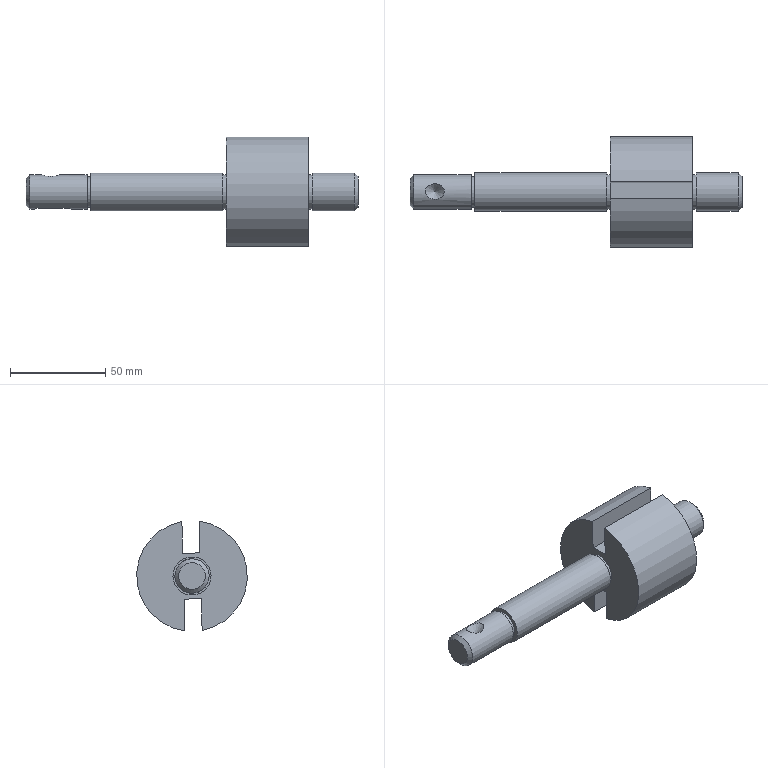Component | NX | ROTOR_SHAFT | 1 solid | 30 faces | volume 138670 mm3 | plane 17 | cylinder 10 | cone 3 | commonest cylinder face diameters 18 x3 58 x2 20 x2 6 x2 16 x1